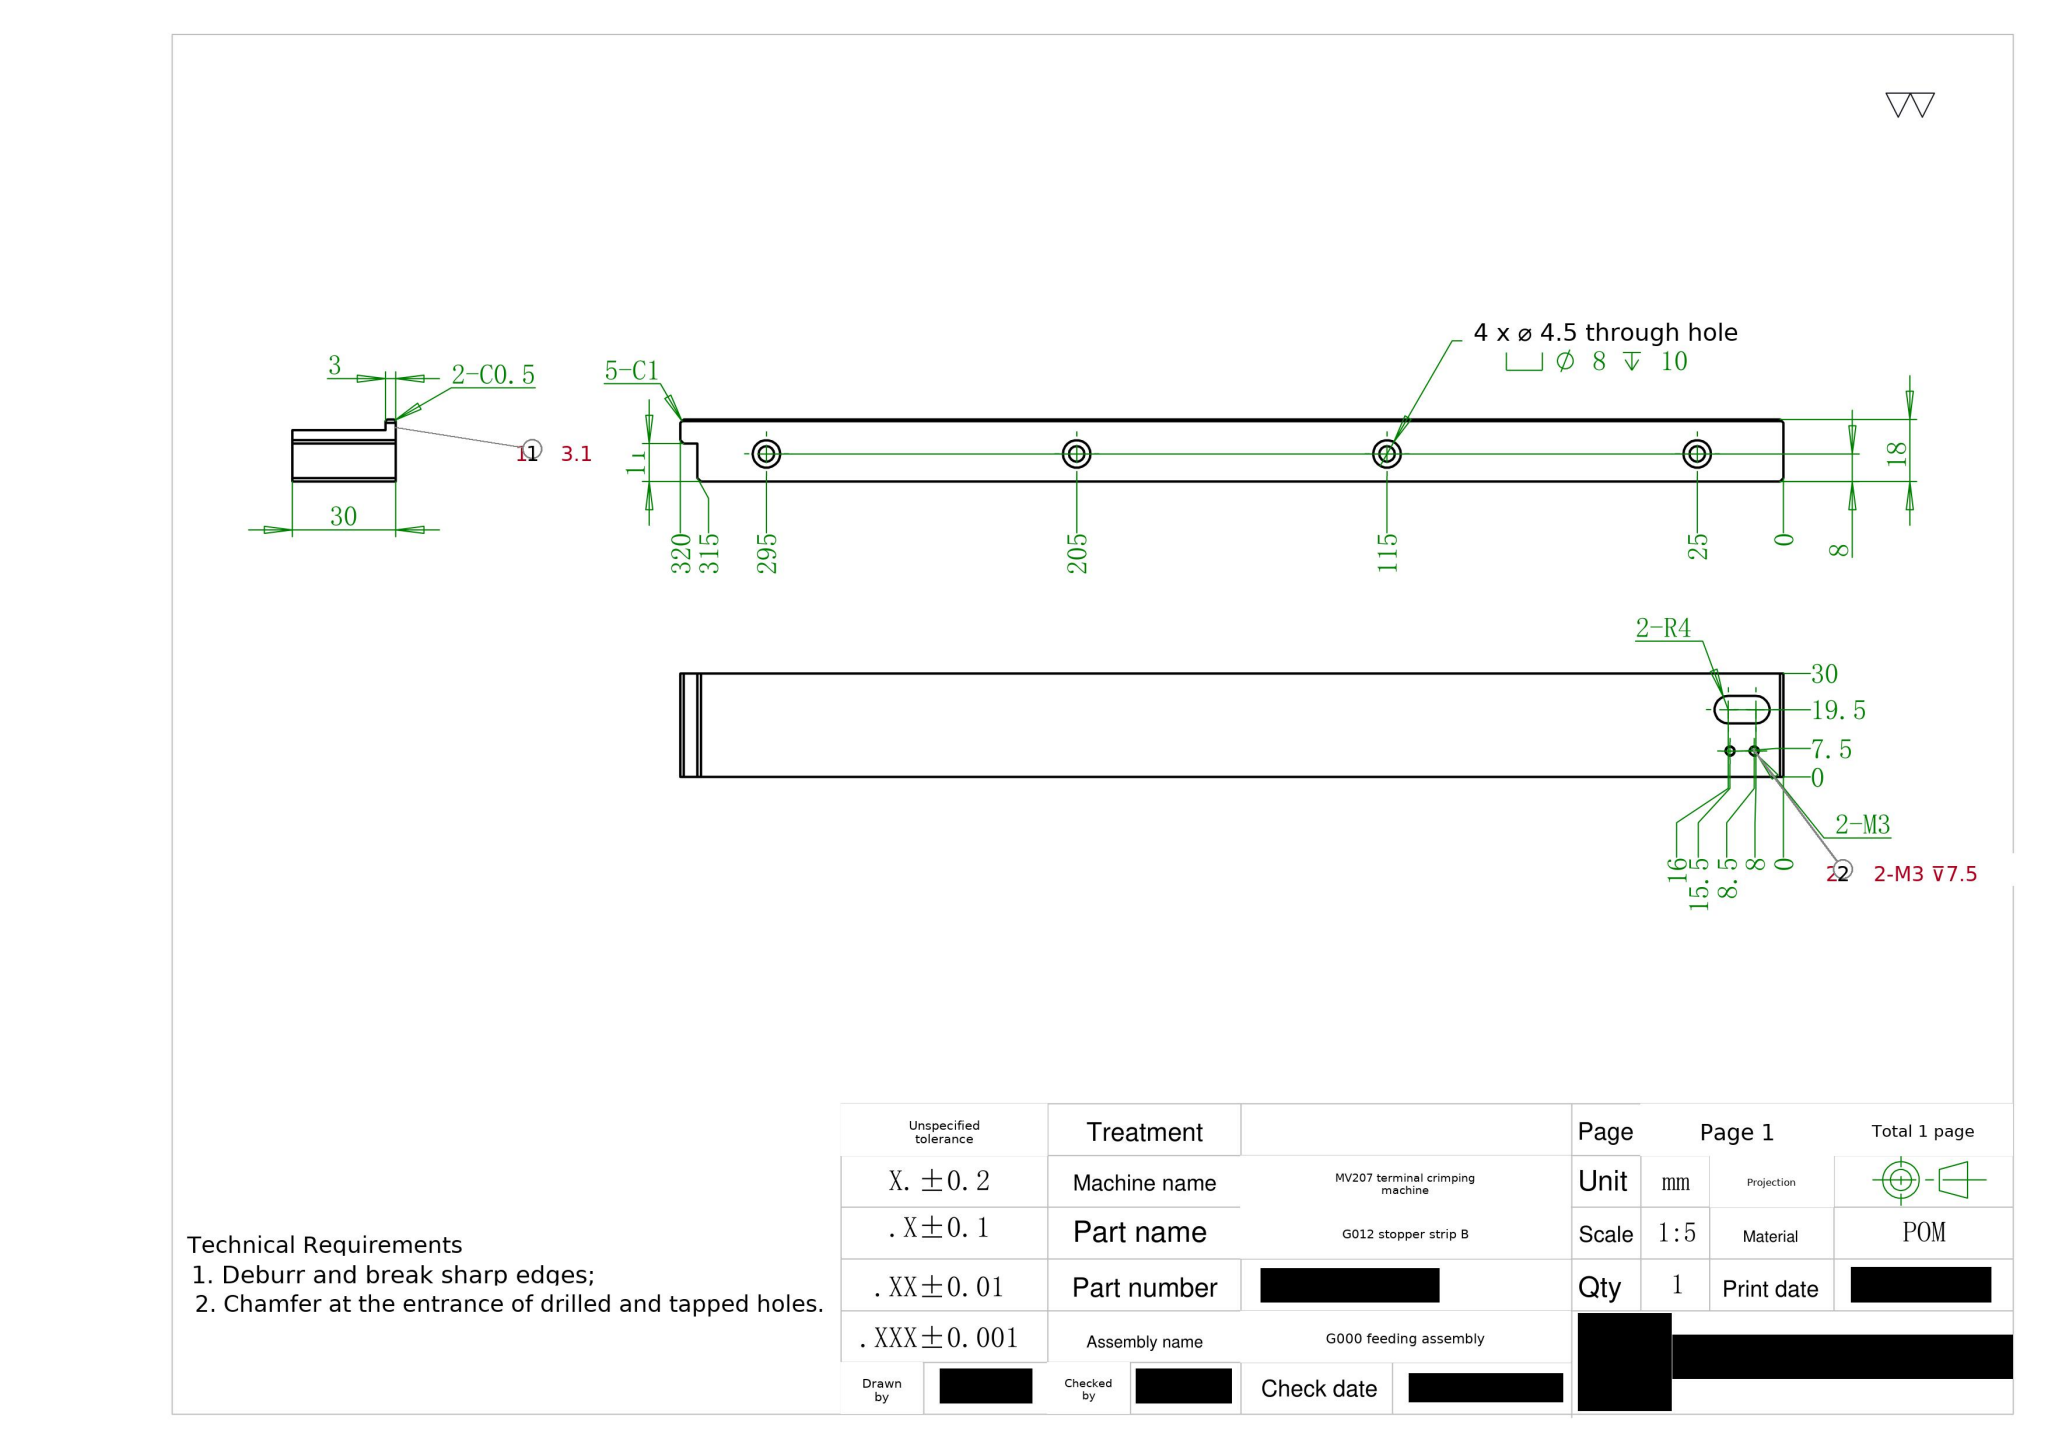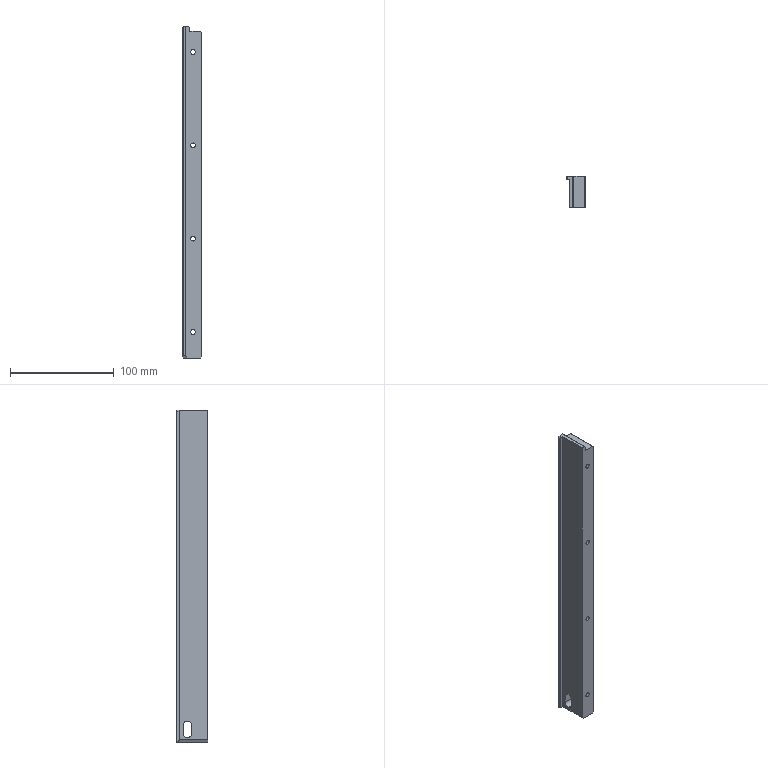Part | SolidWorks | mm | material POM | 1 solid | 52 faces | box 18 x 30 x 320 mm | volume 139142 mm3 | plane 25 | cylinder 23 | cone 4 | commonest cylinder face diameters 8 x11 4.5 x8 2.5 x4
build123d program:
from build123d import *
from OCP.BRepFilletAPI import BRepFilletAPI_MakeChamfer

# Parameters (mm, degrees)
BOSS_EXTRUDE1_DEPTH                             = 320
M3_TAPPED_HOLE1_D                               = 2.5
M3_TAPPED_HOLE1_DEPTH                           = 7.5
M3_TAPPED_HOLE1_TIP                             = 0.7511
M4_HEX_SOCKET_HEAD_CAP_SCREW_CBORE1_D           = 4.5
M4_HEX_SOCKET_HEAD_CAP_SCREW_CBORE1_CBORE_D     = 8
M4_HEX_SOCKET_HEAD_CAP_SCREW_CBORE1_CBORE_DEPTH = 10
SKETCH7_W                                       = 11
SKETCH7_H                                       = 5
CUT_EXTRUDE2_DEPTH                              = 322.907
CUT_EXTRUDE4_DEPTH                              = 322.907
CHAMFER1_SIZE                                   = 0.5
CHAMFER2_SIZE                                   = 2
CHAMFER2_SIZE2                                  = 1.155
CHAMFER3_SIZE                                   = 1


with BuildPart() as part:
    # Sketch1 → Boss-Extrude1 (new body)
    with BuildSketch(Plane.XY):
        Polygon((0, 0), (0, 30), (-18, 30), (-18, 27), (-14.9, 27), (-14.9, 0), align=None)
    extrude(amount=BOSS_EXTRUDE1_DEPTH)

    # M3 Tapped Hole1
    with Locations(Plane(origin=(0, 0, 0), x_dir=(0, 0, -1), z_dir=(1, 0, 0))):
        with Locations((-15.5, 7.5), (-8.5, 7.5)):
            Hole(M3_TAPPED_HOLE1_D / 2, depth=M3_TAPPED_HOLE1_DEPTH)
            with Locations((0, 0, -(M3_TAPPED_HOLE1_DEPTH + M3_TAPPED_HOLE1_TIP / 2))):  # 118° drill point
                Cone(0, M3_TAPPED_HOLE1_D / 2, M3_TAPPED_HOLE1_TIP, mode=Mode.SUBTRACT)

    # M4 Hex Socket Head Cap Screw CBORE1 (through all)
    with Locations(Plane(origin=(0, 30, 0), x_dir=(1, 0, 0), z_dir=(0, 1, 0))):
        with Locations((-8, -25), (-8, -115), (-8, -205), (-8, -295)):
            CounterBoreHole(M4_HEX_SOCKET_HEAD_CAP_SCREW_CBORE1_D / 2, M4_HEX_SOCKET_HEAD_CAP_SCREW_CBORE1_CBORE_D / 2, M4_HEX_SOCKET_HEAD_CAP_SCREW_CBORE1_CBORE_DEPTH)

    # Sketch7 → Cut-Extrude2 (cut, through all)
    with BuildSketch(Plane(origin=(0, 30, 0), x_dir=(1, 0, 0), z_dir=(0, 1, 0))):
        with Locations((-5.5, -317.5)):
            Rectangle(SKETCH7_W, SKETCH7_H)
    extrude(amount=-CUT_EXTRUDE2_DEPTH, mode=Mode.SUBTRACT)

    # Sketch9 → Cut-Extrude4 (cut, through all)
    with BuildSketch(Plane(origin=(0, 0, 0), x_dir=(0, 0, -1), z_dir=(1, 0, 0))):
        with BuildLine():
            Line((-16, 23.5), (-8, 23.5))
            ThreePointArc((-8, 23.5), (-4, 19.5), (-8, 15.5))
            Line((-8, 15.5), (-16, 15.5))
            ThreePointArc((-16, 15.5), (-20, 19.5), (-16, 23.5))
        make_face()
    extrude(amount=-CUT_EXTRUDE4_DEPTH, mode=Mode.SUBTRACT)

    # Chamfer1
    chamfer1_edges = [part.edges().sort_by_distance(p)[0] for p in [
        (-18, 27, 160),
        (-18, 30, 160),
    ]]
    chamfer(chamfer1_edges, length=CHAMFER1_SIZE)

    # Chamfer2: one chamfer whose edges measure the first distance from different faces: ONE call of the kernel's chamfer builder (chamfer() names one face for all edges)
    chamfer2_edges_1 = [part.edges().sort_by_distance(p)[0] for p in [
        (-14.9, 13.5, 0),
    ]]
    chamfer2_side_1 = [part.faces().sort_by_distance(p)[0] for p in [
        (-14.9, 13.42, 161.984),
    ]]
    chamfer2_edges_2 = [part.edges().sort_by_distance(p)[0] for p in [
        (-16.2, 27, 0),
    ]]
    chamfer2_side_2 = [part.faces().sort_by_distance(p)[0] for p in [
        (-16.2, 27, 160),
    ]]
    chamfer2 = BRepFilletAPI_MakeChamfer(part.part.solid().wrapped)
    for e in chamfer2_edges_1:
        chamfer2.Add(CHAMFER2_SIZE, CHAMFER2_SIZE2, e.wrapped, chamfer2_side_1[0].wrapped)  # the first distance lies on this face
    for e in chamfer2_edges_2:
        chamfer2.Add(CHAMFER2_SIZE, CHAMFER2_SIZE2, e.wrapped, chamfer2_side_2[0].wrapped)  # the first distance lies on this face
    add(Compound.cast(chamfer2.Shape()), mode=Mode.REPLACE)

    # Chamfer3
    chamfer3_edges = [part.edges().sort_by_distance(p)[0] for p in [
        (-18, 28.827, 0),
        (0, 15, 0),
        (-18, 28.5, 320),
        (0, 15, 315),
        (-11, 15, 320),
    ]]
    chamfer(chamfer3_edges, length=CHAMFER3_SIZE)


solid = part.part